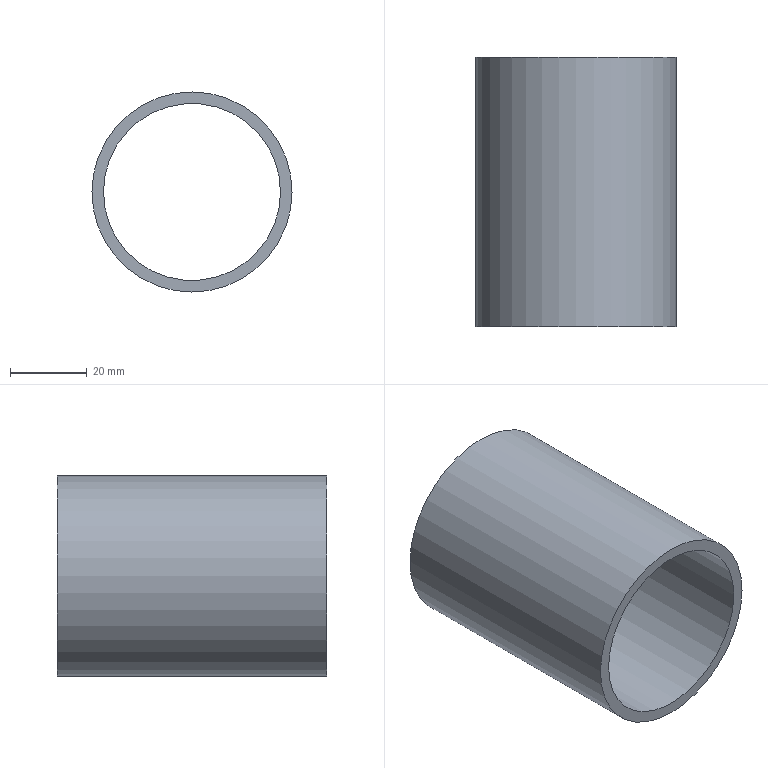Component | NX | MASTER_ROD_BEARING | 1 solid | 4 faces | box 52 x 70 x 52 mm | volume 32327 mm3 | cylinder 2 | plane 2 | commonest cylinder face diameters 52 x1 46 x1
STEP:
#1=CARTESIAN_POINT('',(0.,0.,0.));
#2=DIRECTION('',(0.,0.,1.));
#3=DIRECTION('',(1.,0.,0.));
#4=AXIS2_PLACEMENT_3D('',#1,#2,#3);
#5=CARTESIAN_POINT('',(28.69,-35.,0.9588));
#6=VERTEX_POINT('',#5);
#7=CARTESIAN_POINT('',(2.691,-35.,1.07));
#8=DIRECTION('',(0.,-1.,0.));
#9=DIRECTION('',(1.,0.,-0.00428));
#10=AXIS2_PLACEMENT_3D('',#7,#8,#9);
#11=CIRCLE('',#10,26.);
#12=CARTESIAN_POINT('',(2.691,-35.,1.07));
#13=DIRECTION('',(0.,1.,0.));
#14=DIRECTION('',(-1.,0.,0.00428));
#15=AXIS2_PLACEMENT_3D('',#12,#13,#14);
#16=CYLINDRICAL_SURFACE('',#15,26.);
#17=CARTESIAN_POINT('',(9.425,0.));
#18=DIRECTION('',(-1.,0.));
#19=VECTOR('',#18,1.);
#20=LINE('',#17,#19);
#21=(GEOMETRIC_REPRESENTATION_CONTEXT(2)PARAMETRIC_REPRESENTATION_CONTEXT()REPRESENTATION_CONTEXT('',''));
#22=DEFINITIONAL_REPRESENTATION('',(#20),#21);
#23=PCURVE('',#16,#22);
#24=CARTESIAN_POINT('',(2.691,-35.,1.07));
#25=DIRECTION('',(0.,-1.,0.));
#26=DIRECTION('',(1.,0.,-0.00428));
#27=AXIS2_PLACEMENT_3D('',#24,#25,#26);
#28=PLANE('',#27);
#29=CARTESIAN_POINT('',(0.,0.));
#30=DIRECTION('',(1.,0.));
#31=AXIS2_PLACEMENT_2D('',#29,#30);
#32=CIRCLE('',#31,26.);
#33=(GEOMETRIC_REPRESENTATION_CONTEXT(2)PARAMETRIC_REPRESENTATION_CONTEXT()REPRESENTATION_CONTEXT('',''));
#34=DEFINITIONAL_REPRESENTATION('',(#32),#33);
#35=PCURVE('',#28,#34);
#36=SURFACE_CURVE('',#11,(#23,#35),.PCURVE_S1.);
#37=EDGE_CURVE('',#6,#6,#36,.T.);
#38=ORIENTED_EDGE('',*,*,#37,.F.);
#39=CARTESIAN_POINT('',(28.69,35.,0.9588));
#40=VERTEX_POINT('',#39);
#41=CARTESIAN_POINT('',(28.69,-35.,0.9588));
#42=CARTESIAN_POINT('',(28.69,35.,0.9588));
#43=B_SPLINE_CURVE_WITH_KNOTS('',1,(#41,#42),.UNSPECIFIED.,.F.,.F.,(2,2),(0.,70.),.PIECEWISE_BEZIER_KNOTS.);
#44=CARTESIAN_POINT('',(9.425,0.));
#45=DIRECTION('',(0.,1.));
#46=VECTOR('',#45,1.);
#47=LINE('',#44,#46);
#48=(GEOMETRIC_REPRESENTATION_CONTEXT(2)PARAMETRIC_REPRESENTATION_CONTEXT()REPRESENTATION_CONTEXT('',''));
#49=DEFINITIONAL_REPRESENTATION('',(#47),#48);
#50=PCURVE('',#16,#49);
#51=CARTESIAN_POINT('',(3.142,0.));
#52=DIRECTION('',(0.,1.));
#53=VECTOR('',#52,1.);
#54=LINE('',#51,#53);
#55=(GEOMETRIC_REPRESENTATION_CONTEXT(2)PARAMETRIC_REPRESENTATION_CONTEXT()REPRESENTATION_CONTEXT('',''));
#56=DEFINITIONAL_REPRESENTATION('',(#54),#55);
#57=PCURVE('',#16,#56);
#58=SEAM_CURVE('',#43,(#50,#57),.PCURVE_S1.);
#59=EDGE_CURVE('',#6,#40,#58,.T.);
#60=ORIENTED_EDGE('',*,*,#59,.T.);
#61=CARTESIAN_POINT('',(2.691,35.,1.07));
#62=DIRECTION('',(0.,-1.,0.));
#63=DIRECTION('',(1.,0.,-0.00428));
#64=AXIS2_PLACEMENT_3D('',#61,#62,#63);
#65=CIRCLE('',#64,26.);
#66=CARTESIAN_POINT('',(9.425,70.));
#67=DIRECTION('',(-1.,0.));
#68=VECTOR('',#67,1.);
#69=LINE('',#66,#68);
#70=(GEOMETRIC_REPRESENTATION_CONTEXT(2)PARAMETRIC_REPRESENTATION_CONTEXT()REPRESENTATION_CONTEXT('',''));
#71=DEFINITIONAL_REPRESENTATION('',(#69),#70);
#72=PCURVE('',#16,#71);
#73=CARTESIAN_POINT('',(2.691,35.,1.07));
#74=DIRECTION('',(0.,-1.,0.));
#75=DIRECTION('',(1.,0.,-0.00428));
#76=AXIS2_PLACEMENT_3D('',#73,#74,#75);
#77=PLANE('',#76);
#78=CARTESIAN_POINT('',(0.,0.));
#79=DIRECTION('',(1.,0.));
#80=AXIS2_PLACEMENT_2D('',#78,#79);
#81=CIRCLE('',#80,26.);
#82=(GEOMETRIC_REPRESENTATION_CONTEXT(2)PARAMETRIC_REPRESENTATION_CONTEXT()REPRESENTATION_CONTEXT('',''));
#83=DEFINITIONAL_REPRESENTATION('',(#81),#82);
#84=PCURVE('',#77,#83);
#85=SURFACE_CURVE('',#65,(#72,#84),.PCURVE_S1.);
#86=EDGE_CURVE('',#40,#40,#85,.T.);
#87=ORIENTED_EDGE('',*,*,#86,.T.);
#88=ORIENTED_EDGE('',*,*,#59,.F.);
#89=EDGE_LOOP('',(#38,#60,#87,#88));
#90=FACE_BOUND('',#89,.T.);
#91=ADVANCED_FACE('',(#90),#16,.T.);
#92=CARTESIAN_POINT('',(25.691,-35.,0.9716));
#93=VERTEX_POINT('',#92);
#94=CARTESIAN_POINT('',(2.691,-35.,1.07));
#95=DIRECTION('',(0.,-1.,0.));
#96=DIRECTION('',(1.,0.,-0.00428));
#97=AXIS2_PLACEMENT_3D('',#94,#95,#96);
#98=CIRCLE('',#97,23.);
#99=CARTESIAN_POINT('',(2.691,-35.,1.07));
#100=DIRECTION('',(0.,1.,0.));
#101=DIRECTION('',(-1.,0.,0.00428));
#102=AXIS2_PLACEMENT_3D('',#99,#100,#101);
#103=CYLINDRICAL_SURFACE('',#102,23.);
#104=CARTESIAN_POINT('',(9.425,0.));
#105=DIRECTION('',(-1.,0.));
#106=VECTOR('',#105,1.);
#107=LINE('',#104,#106);
#108=(GEOMETRIC_REPRESENTATION_CONTEXT(2)PARAMETRIC_REPRESENTATION_CONTEXT()REPRESENTATION_CONTEXT('',''));
#109=DEFINITIONAL_REPRESENTATION('',(#107),#108);
#110=PCURVE('',#103,#109);
#111=CARTESIAN_POINT('',(0.,0.));
#112=DIRECTION('',(1.,-0.));
#113=AXIS2_PLACEMENT_2D('',#111,#112);
#114=CIRCLE('',#113,23.);
#115=(GEOMETRIC_REPRESENTATION_CONTEXT(2)PARAMETRIC_REPRESENTATION_CONTEXT()REPRESENTATION_CONTEXT('',''));
#116=DEFINITIONAL_REPRESENTATION('',(#114),#115);
#117=PCURVE('',#28,#116);
#118=SURFACE_CURVE('',#98,(#110,#117),.PCURVE_S1.);
#119=EDGE_CURVE('',#93,#93,#118,.T.);
#120=ORIENTED_EDGE('',*,*,#119,.F.);
#121=CARTESIAN_POINT('',(25.691,35.,0.9716));
#122=VERTEX_POINT('',#121);
#123=CARTESIAN_POINT('',(25.691,-35.,0.9716));
#124=CARTESIAN_POINT('',(25.691,35.,0.9716));
#125=B_SPLINE_CURVE_WITH_KNOTS('',1,(#123,#124),.UNSPECIFIED.,.F.,.F.,(2,2),(0.,70.),.PIECEWISE_BEZIER_KNOTS.);
#126=CARTESIAN_POINT('',(9.425,0.));
#127=DIRECTION('',(0.,1.));
#128=VECTOR('',#127,1.);
#129=LINE('',#126,#128);
#130=(GEOMETRIC_REPRESENTATION_CONTEXT(2)PARAMETRIC_REPRESENTATION_CONTEXT()REPRESENTATION_CONTEXT('',''));
#131=DEFINITIONAL_REPRESENTATION('',(#129),#130);
#132=PCURVE('',#103,#131);
#133=CARTESIAN_POINT('',(3.142,0.));
#134=DIRECTION('',(0.,1.));
#135=VECTOR('',#134,1.);
#136=LINE('',#133,#135);
#137=(GEOMETRIC_REPRESENTATION_CONTEXT(2)PARAMETRIC_REPRESENTATION_CONTEXT()REPRESENTATION_CONTEXT('',''));
#138=DEFINITIONAL_REPRESENTATION('',(#136),#137);
#139=PCURVE('',#103,#138);
#140=SEAM_CURVE('',#125,(#132,#139),.PCURVE_S1.);
#141=EDGE_CURVE('',#93,#122,#140,.T.);
#142=ORIENTED_EDGE('',*,*,#141,.T.);
#143=CARTESIAN_POINT('',(2.691,35.,1.07));
#144=DIRECTION('',(0.,-1.,0.));
#145=DIRECTION('',(1.,0.,-0.00428));
#146=AXIS2_PLACEMENT_3D('',#143,#144,#145);
#147=CIRCLE('',#146,23.);
#148=CARTESIAN_POINT('',(9.425,70.));
#149=DIRECTION('',(-1.,0.));
#150=VECTOR('',#149,1.);
#151=LINE('',#148,#150);
#152=(GEOMETRIC_REPRESENTATION_CONTEXT(2)PARAMETRIC_REPRESENTATION_CONTEXT()REPRESENTATION_CONTEXT('',''));
#153=DEFINITIONAL_REPRESENTATION('',(#151),#152);
#154=PCURVE('',#103,#153);
#155=CARTESIAN_POINT('',(0.,0.));
#156=DIRECTION('',(1.,-0.));
#157=AXIS2_PLACEMENT_2D('',#155,#156);
#158=CIRCLE('',#157,23.);
#159=(GEOMETRIC_REPRESENTATION_CONTEXT(2)PARAMETRIC_REPRESENTATION_CONTEXT()REPRESENTATION_CONTEXT('',''));
#160=DEFINITIONAL_REPRESENTATION('',(#158),#159);
#161=PCURVE('',#77,#160);
#162=SURFACE_CURVE('',#147,(#154,#161),.PCURVE_S1.);
#163=EDGE_CURVE('',#122,#122,#162,.T.);
#164=ORIENTED_EDGE('',*,*,#163,.T.);
#165=ORIENTED_EDGE('',*,*,#141,.F.);
#166=EDGE_LOOP('',(#120,#142,#164,#165));
#167=FACE_BOUND('',#166,.F.);
#168=ADVANCED_FACE('',(#167),#103,.F.);
#169=ORIENTED_EDGE('',*,*,#37,.T.);
#170=EDGE_LOOP('',(#169));
#171=FACE_BOUND('',#170,.T.);
#172=ORIENTED_EDGE('',*,*,#119,.F.);
#173=EDGE_LOOP('',(#172));
#174=FACE_BOUND('',#173,.T.);
#175=ADVANCED_FACE('',(#171,#174),#28,.T.);
#176=ORIENTED_EDGE('',*,*,#86,.F.);
#177=EDGE_LOOP('',(#176));
#178=FACE_BOUND('',#177,.T.);
#179=ORIENTED_EDGE('',*,*,#163,.T.);
#180=EDGE_LOOP('',(#179));
#181=FACE_BOUND('',#180,.T.);
#182=ADVANCED_FACE('',(#178,#181),#77,.F.);
#183=CLOSED_SHELL('',(#91,#168,#175,#182));
#184=MANIFOLD_SOLID_BREP('',#183);
#185=(LENGTH_UNIT()NAMED_UNIT(*)SI_UNIT(.MILLI.,.METRE.));
#186=UNCERTAINTY_MEASURE_WITH_UNIT(LENGTH_MEASURE(0.00001),#185,'','');
#187=(NAMED_UNIT(*)PLANE_ANGLE_UNIT()SI_UNIT($,.RADIAN.));
#188=(NAMED_UNIT(*)SI_UNIT($,.STERADIAN.)SOLID_ANGLE_UNIT());
#189=(GEOMETRIC_REPRESENTATION_CONTEXT(3)GLOBAL_UNCERTAINTY_ASSIGNED_CONTEXT((#186))GLOBAL_UNIT_ASSIGNED_CONTEXT((#185,#187,#188))REPRESENTATION_CONTEXT('',''));
#190=ADVANCED_BREP_SHAPE_REPRESENTATION('',(#4,#184),#189);